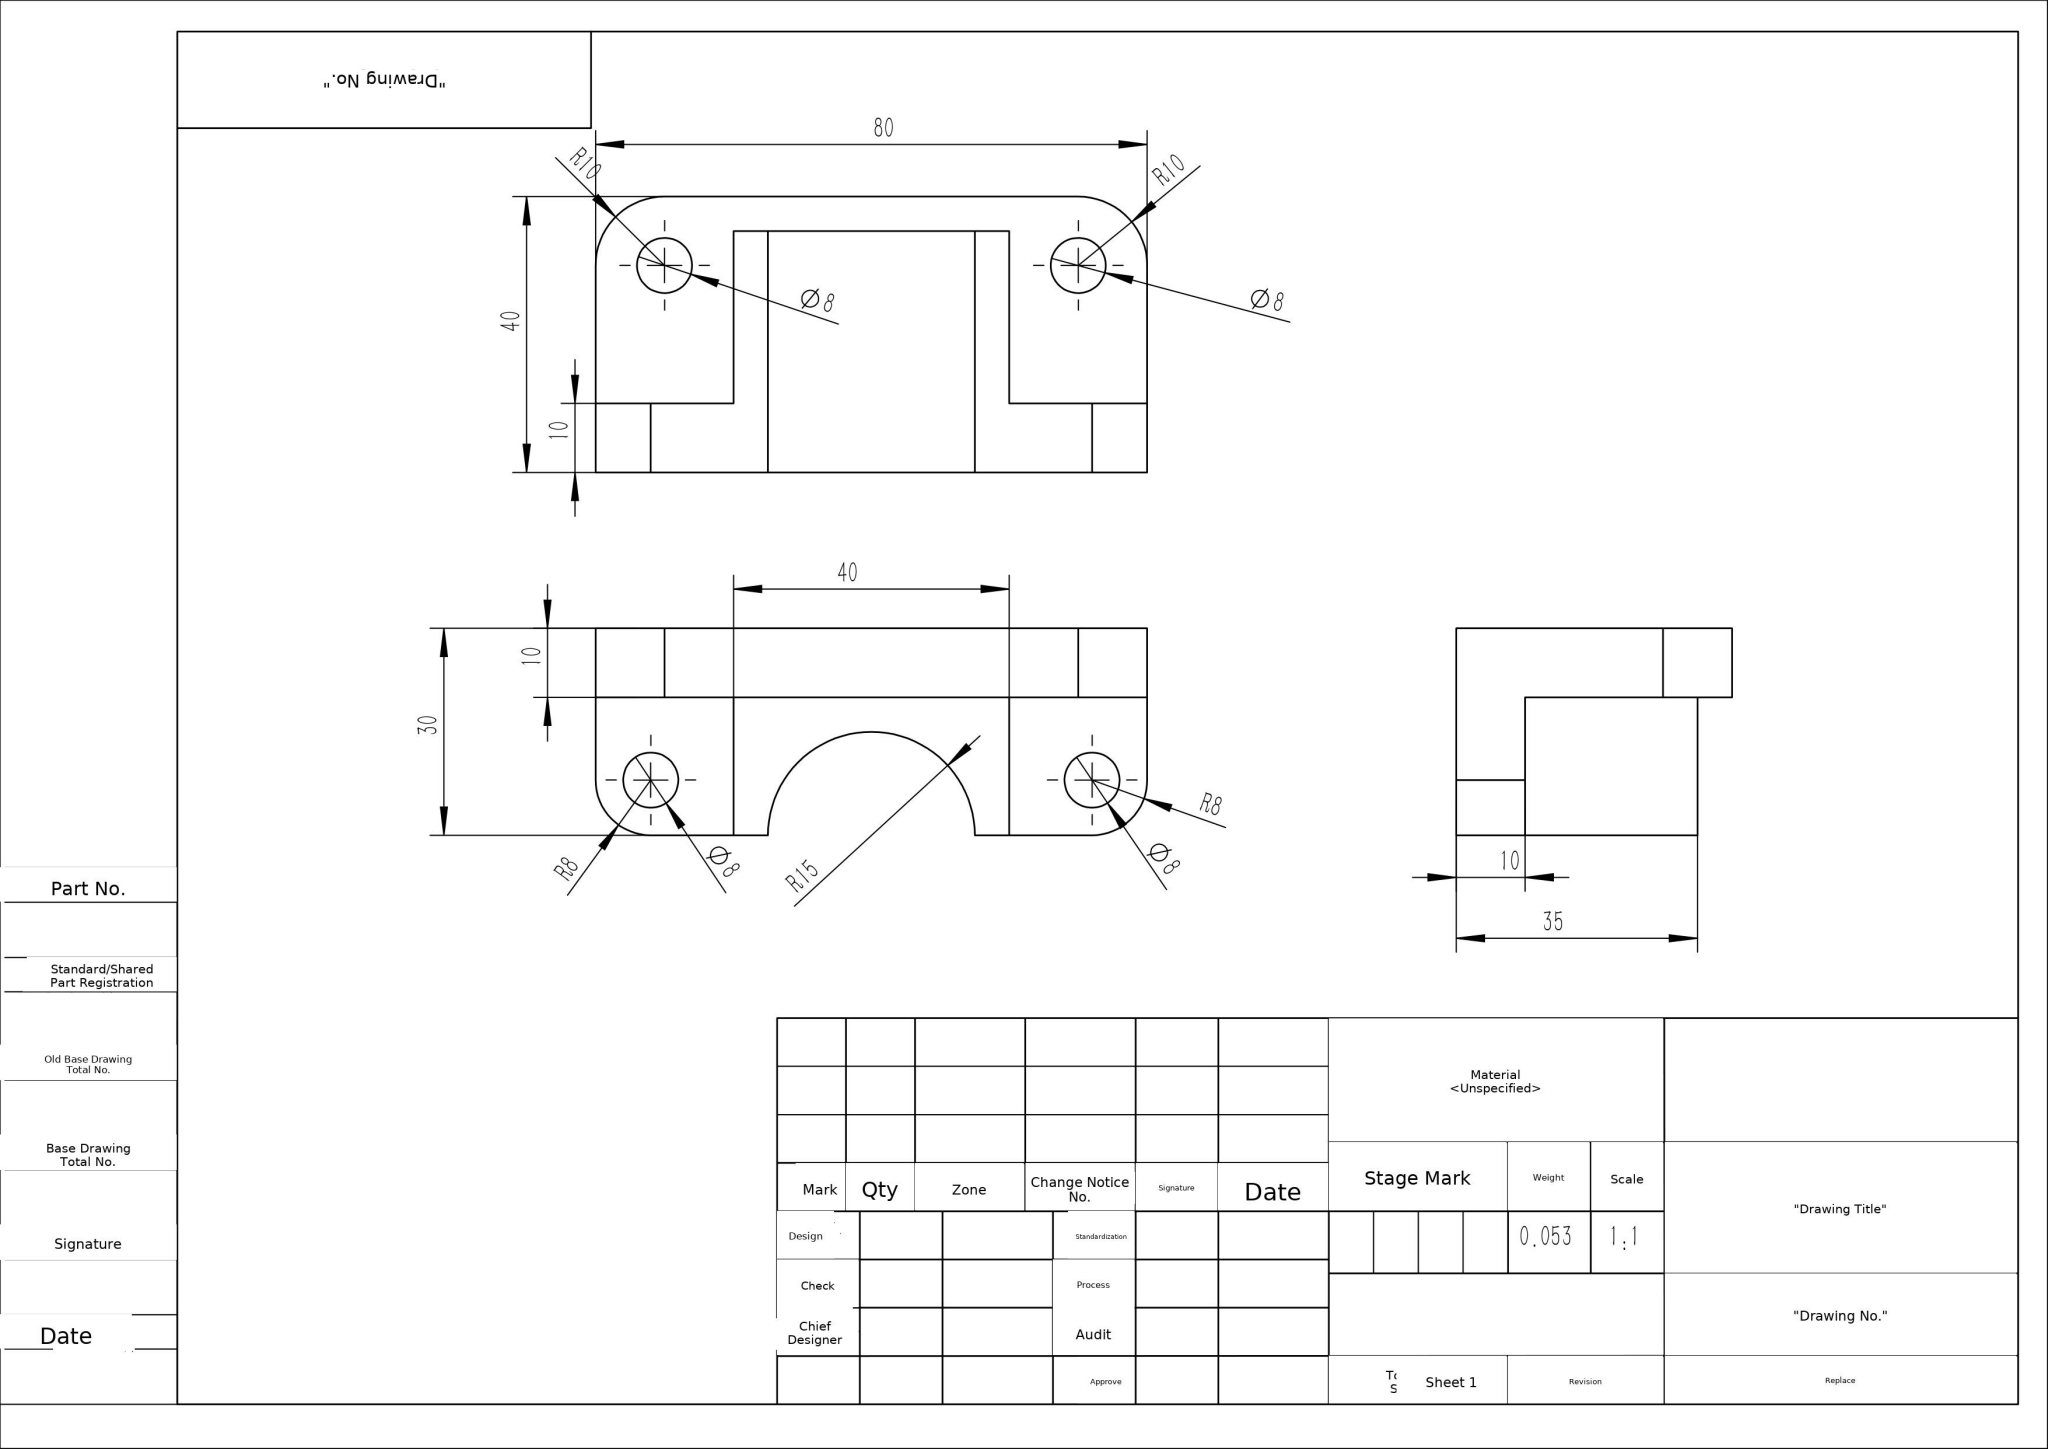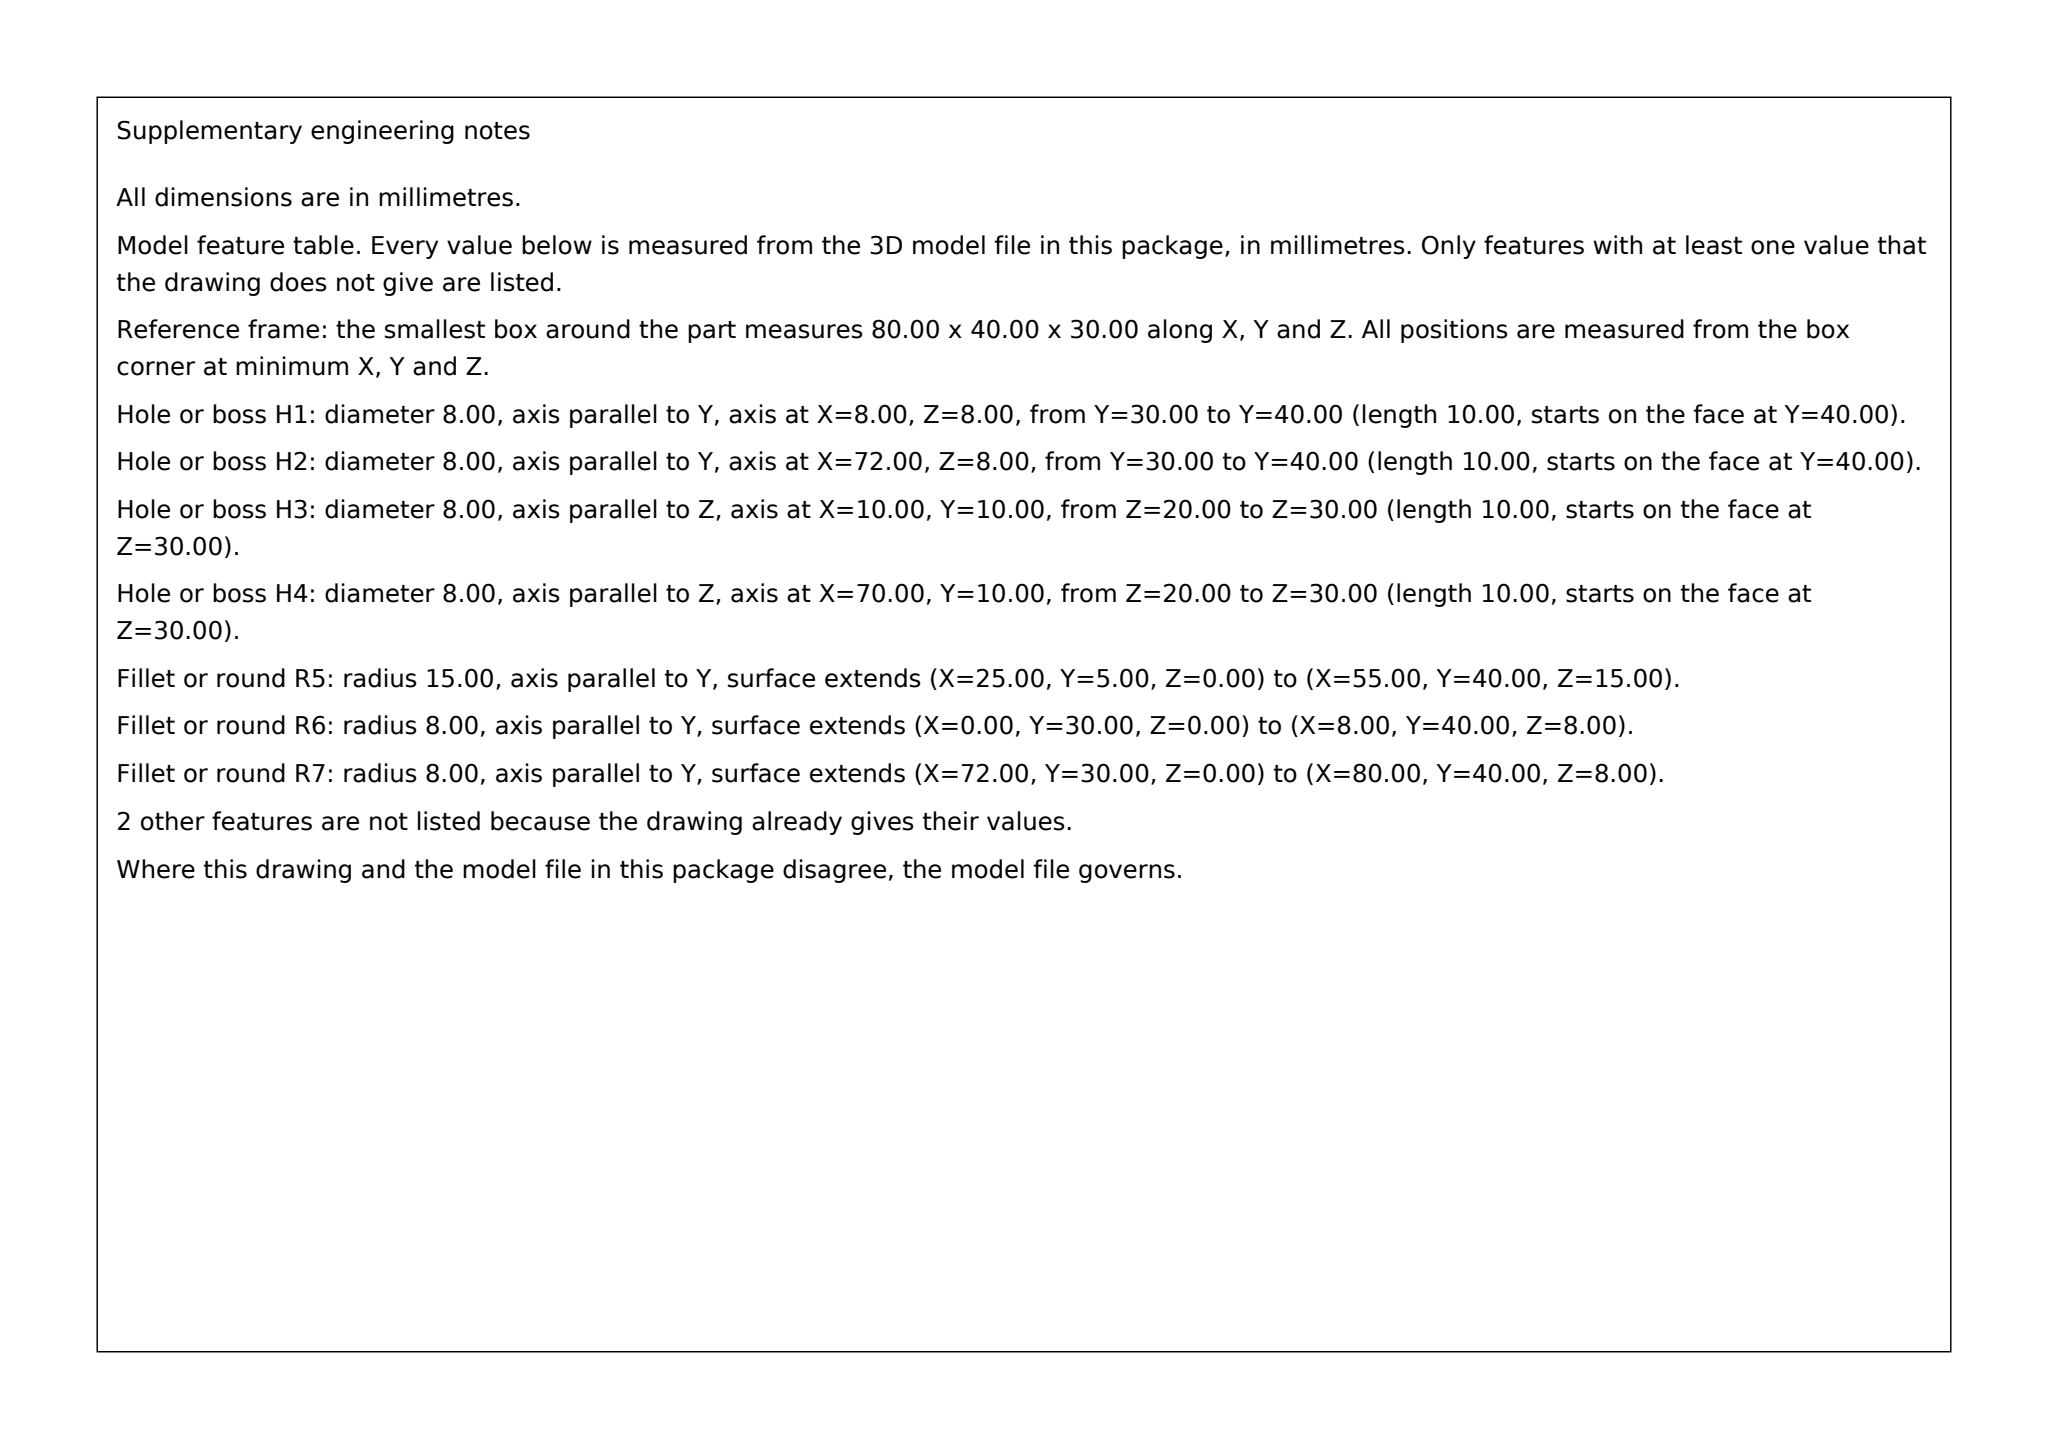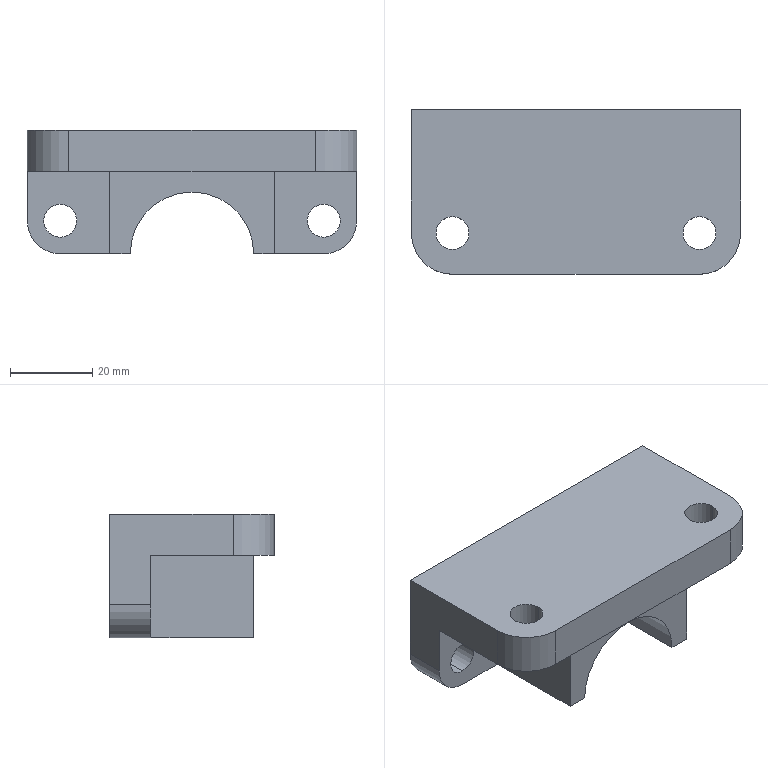Part | SolidWorks | mm | 1 solid | 27 faces | box 80 x 40 x 30 mm | volume 52915 mm3 | cylinder 14 | plane 13 | commonest cylinder face diameters 8 x8 30 x2 20 x2 16 x2
build123d program:
from build123d import *

# Parameters (mm, degrees)
SKETCH1_R           = 4
BOSS_EXTRUDE1_DEPTH = 10
SKETCH2_R           = 4
BOSS_EXTRUDE2_DEPTH = 10
BOSS_EXTRUDE3_DEPTH = 25


with BuildPart() as part:
    # Sketch1 → Boss-Extrude1 (new body)
    with BuildSketch(Plane.XY):
        with BuildLine():
            Line((-30, -20), (30, -20))
            ThreePointArc((30, -20), (37.071, -17.071), (40, -10))
            Line((40, -10), (40, 20))
            Line((40, 20), (-40, 20))
            Line((-40, 20), (-40, -10))
            ThreePointArc((-40, -10), (-37.071, -17.071), (-30, -20))
        make_face()
        with Locations((30, -10)):
            Circle(SKETCH1_R, mode=Mode.SUBTRACT)
        with Locations((-30, -10)):
            Circle(SKETCH1_R, mode=Mode.SUBTRACT)
    extrude(amount=BOSS_EXTRUDE1_DEPTH)

    # Sketch2 → Boss-Extrude2 (add)
    with BuildSketch(Plane(origin=(0, 20, 0), x_dir=(1, 0, 0), z_dir=(0, 1, 0))):
        with BuildLine():
            Line((15, 20), (32, 20))
            ThreePointArc((32, 20), (37.657, 17.657), (40, 12))
            Line((40, 12), (40, 0))
            Line((40, 0), (-40, 0))
            Line((-40, 0), (-40, 12))
            ThreePointArc((-40, 12), (-37.657, 17.657), (-32, 20))
            Line((-32, 20), (-15, 20))
            ThreePointArc((-15, 20), (0, 5), (15, 20))
        make_face()
        with Locations(Location((-32, 12, 0), (0, 0, 270))):
            Circle(SKETCH2_R, mode=Mode.SUBTRACT)
        with Locations(Location((32, 12, 0), (0, 0, 270))):
            Circle(SKETCH2_R, mode=Mode.SUBTRACT)
    extrude(amount=-BOSS_EXTRUDE2_DEPTH)

    # Sketch3 → Boss-Extrude3 (add)
    with BuildSketch(Plane.XZ.offset(-10)):
        with BuildLine():
            Line((-15, -20), (-20, -20))
            Line((-20, -20), (-20, 0))
            Line((-20, 0), (20, 0))
            Line((20, 0), (20, -20))
            Line((20, -20), (15, -20))
            ThreePointArc((15, -20), (0, -5), (-15, -20))
        make_face()
    extrude(amount=BOSS_EXTRUDE3_DEPTH)


solid = part.part
STEP:
#1=CARTESIAN_POINT('',(32.,10.,-16.));
#2=VERTEX_POINT('',#1);
#3=CARTESIAN_POINT('',(32.,10.,-8.));
#4=VERTEX_POINT('',#3);
#5=CARTESIAN_POINT('',(32.,10.,-12.));
#6=DIRECTION('',(0.,1.,0.));
#7=DIRECTION('',(0.,0.,1.));
#8=AXIS2_PLACEMENT_3D('',#5,#6,#7);
#9=CIRCLE('',#8,4.);
#10=EDGE_CURVE('',#2,#4,#9,.T.);
#11=ORIENTED_EDGE('',*,*,#10,.F.);
#12=CARTESIAN_POINT('',(32.,20.,-16.));
#13=VERTEX_POINT('',#12);
#14=CARTESIAN_POINT('',(32.,10.,-16.));
#15=DIRECTION('',(0.,1.,0.));
#16=VECTOR('',#15,1000.);
#17=LINE('',#14,#16);
#18=EDGE_CURVE('',#2,#13,#17,.T.);
#19=ORIENTED_EDGE('',*,*,#18,.T.);
#20=CARTESIAN_POINT('',(32.,20.,-8.));
#21=VERTEX_POINT('',#20);
#22=CARTESIAN_POINT('',(32.,20.,-12.));
#23=DIRECTION('',(0.,1.,0.));
#24=DIRECTION('',(0.,0.,1.));
#25=AXIS2_PLACEMENT_3D('',#22,#23,#24);
#26=CIRCLE('',#25,4.);
#27=EDGE_CURVE('',#13,#21,#26,.T.);
#28=ORIENTED_EDGE('',*,*,#27,.T.);
#29=CARTESIAN_POINT('',(32.,10.,-8.));
#30=DIRECTION('',(0.,1.,0.));
#31=VECTOR('',#30,1000.);
#32=LINE('',#29,#31);
#33=EDGE_CURVE('',#4,#21,#32,.T.);
#34=ORIENTED_EDGE('',*,*,#33,.F.);
#35=EDGE_LOOP('',(#11,#19,#28,#34));
#36=FACE_OUTER_BOUND('',#35,.T.);
#37=CARTESIAN_POINT('',(32.,10.,-12.));
#38=DIRECTION('',(0.,1.,0.));
#39=DIRECTION('',(0.,0.,1.));
#40=AXIS2_PLACEMENT_3D('',#37,#38,#39);
#41=CYLINDRICAL_SURFACE('',#40,4.);
#42=ADVANCED_FACE('',(#36),#41,.F.);
#43=CARTESIAN_POINT('',(-32.,10.,-16.));
#44=VERTEX_POINT('',#43);
#45=CARTESIAN_POINT('',(-32.,10.,-8.));
#46=VERTEX_POINT('',#45);
#47=CARTESIAN_POINT('',(-32.,10.,-12.));
#48=DIRECTION('',(0.,1.,0.));
#49=DIRECTION('',(0.,0.,1.));
#50=AXIS2_PLACEMENT_3D('',#47,#48,#49);
#51=CIRCLE('',#50,4.);
#52=EDGE_CURVE('',#44,#46,#51,.T.);
#53=ORIENTED_EDGE('',*,*,#52,.F.);
#54=CARTESIAN_POINT('',(-32.,20.,-16.));
#55=VERTEX_POINT('',#54);
#56=CARTESIAN_POINT('',(-32.,10.,-16.));
#57=DIRECTION('',(0.,1.,0.));
#58=VECTOR('',#57,1000.);
#59=LINE('',#56,#58);
#60=EDGE_CURVE('',#44,#55,#59,.T.);
#61=ORIENTED_EDGE('',*,*,#60,.T.);
#62=CARTESIAN_POINT('',(-32.,20.,-8.));
#63=VERTEX_POINT('',#62);
#64=CARTESIAN_POINT('',(-32.,20.,-12.));
#65=DIRECTION('',(0.,1.,0.));
#66=DIRECTION('',(0.,0.,1.));
#67=AXIS2_PLACEMENT_3D('',#64,#65,#66);
#68=CIRCLE('',#67,4.);
#69=EDGE_CURVE('',#55,#63,#68,.T.);
#70=ORIENTED_EDGE('',*,*,#69,.T.);
#71=CARTESIAN_POINT('',(-32.,10.,-8.));
#72=DIRECTION('',(0.,1.,0.));
#73=VECTOR('',#72,1000.);
#74=LINE('',#71,#73);
#75=EDGE_CURVE('',#46,#63,#74,.T.);
#76=ORIENTED_EDGE('',*,*,#75,.F.);
#77=EDGE_LOOP('',(#53,#61,#70,#76));
#78=FACE_OUTER_BOUND('',#77,.T.);
#79=CARTESIAN_POINT('',(-32.,10.,-12.));
#80=DIRECTION('',(0.,1.,0.));
#81=DIRECTION('',(0.,0.,1.));
#82=AXIS2_PLACEMENT_3D('',#79,#80,#81);
#83=CYLINDRICAL_SURFACE('',#82,4.);
#84=ADVANCED_FACE('',(#78),#83,.F.);
#85=CARTESIAN_POINT('',(-0.,-15.,-5.));
#86=VERTEX_POINT('',#85);
#87=CARTESIAN_POINT('',(15.,-15.,-20.));
#88=VERTEX_POINT('',#87);
#89=CARTESIAN_POINT('',(-0.,-15.,-20.));
#90=DIRECTION('',(0.,1.,0.));
#91=DIRECTION('',(0.,0.,-1.));
#92=AXIS2_PLACEMENT_3D('',#89,#90,#91);
#93=CIRCLE('',#92,15.);
#94=EDGE_CURVE('',#86,#88,#93,.T.);
#95=ORIENTED_EDGE('',*,*,#94,.F.);
#96=CARTESIAN_POINT('',(-0.,20.,-5.));
#97=VERTEX_POINT('',#96);
#98=CARTESIAN_POINT('',(-0.,10.,-5.));
#99=DIRECTION('',(0.,1.,0.));
#100=VECTOR('',#99,1000.);
#101=LINE('',#98,#100);
#102=EDGE_CURVE('',#86,#97,#101,.T.);
#103=ORIENTED_EDGE('',*,*,#102,.T.);
#104=CARTESIAN_POINT('',(15.,20.,-20.));
#105=VERTEX_POINT('',#104);
#106=CARTESIAN_POINT('',(-0.,20.,-20.));
#107=DIRECTION('',(0.,-1.,0.));
#108=DIRECTION('',(0.,0.,1.));
#109=AXIS2_PLACEMENT_3D('',#106,#107,#108);
#110=CIRCLE('',#109,15.);
#111=EDGE_CURVE('',#105,#97,#110,.T.);
#112=ORIENTED_EDGE('',*,*,#111,.F.);
#113=CARTESIAN_POINT('',(15.,10.,-20.));
#114=DIRECTION('',(0.,1.,0.));
#115=VECTOR('',#114,1000.);
#116=LINE('',#113,#115);
#117=EDGE_CURVE('',#88,#105,#116,.T.);
#118=ORIENTED_EDGE('',*,*,#117,.F.);
#119=EDGE_LOOP('',(#95,#103,#112,#118));
#120=FACE_OUTER_BOUND('',#119,.T.);
#121=CARTESIAN_POINT('',(-0.,10.,-20.));
#122=DIRECTION('',(0.,1.,0.));
#123=DIRECTION('',(0.,0.,1.));
#124=AXIS2_PLACEMENT_3D('',#121,#122,#123);
#125=CYLINDRICAL_SURFACE('',#124,15.);
#126=ADVANCED_FACE('',(#120),#125,.F.);
#127=CARTESIAN_POINT('',(-34.,-10.,10.));
#128=VERTEX_POINT('',#127);
#129=CARTESIAN_POINT('',(-26.,-10.,10.));
#130=VERTEX_POINT('',#129);
#131=CARTESIAN_POINT('',(-30.,-10.,10.));
#132=DIRECTION('',(0.,0.,1.));
#133=DIRECTION('',(1.,0.,0.));
#134=AXIS2_PLACEMENT_3D('',#131,#132,#133);
#135=CIRCLE('',#134,4.);
#136=EDGE_CURVE('',#128,#130,#135,.T.);
#137=ORIENTED_EDGE('',*,*,#136,.T.);
#138=CARTESIAN_POINT('',(-26.,-10.,0.));
#139=VERTEX_POINT('',#138);
#140=CARTESIAN_POINT('',(-26.,-10.,10.));
#141=DIRECTION('',(0.,0.,-1.));
#142=VECTOR('',#141,1000.);
#143=LINE('',#140,#142);
#144=EDGE_CURVE('',#130,#139,#143,.T.);
#145=ORIENTED_EDGE('',*,*,#144,.T.);
#146=CARTESIAN_POINT('',(-34.,-10.,0.));
#147=VERTEX_POINT('',#146);
#148=CARTESIAN_POINT('',(-30.,-10.,0.));
#149=DIRECTION('',(0.,0.,1.));
#150=DIRECTION('',(1.,0.,0.));
#151=AXIS2_PLACEMENT_3D('',#148,#149,#150);
#152=CIRCLE('',#151,4.);
#153=EDGE_CURVE('',#147,#139,#152,.T.);
#154=ORIENTED_EDGE('',*,*,#153,.F.);
#155=CARTESIAN_POINT('',(-34.,-10.,10.));
#156=DIRECTION('',(0.,0.,-1.));
#157=VECTOR('',#156,1000.);
#158=LINE('',#155,#157);
#159=EDGE_CURVE('',#128,#147,#158,.T.);
#160=ORIENTED_EDGE('',*,*,#159,.F.);
#161=EDGE_LOOP('',(#137,#145,#154,#160));
#162=FACE_OUTER_BOUND('',#161,.T.);
#163=CARTESIAN_POINT('',(-30.,-10.,10.));
#164=DIRECTION('',(0.,0.,-1.));
#165=DIRECTION('',(-1.,0.,0.));
#166=AXIS2_PLACEMENT_3D('',#163,#164,#165);
#167=CYLINDRICAL_SURFACE('',#166,4.);
#168=ADVANCED_FACE('',(#162),#167,.F.);
#169=CARTESIAN_POINT('',(26.,-10.,10.));
#170=VERTEX_POINT('',#169);
#171=CARTESIAN_POINT('',(34.,-10.,10.));
#172=VERTEX_POINT('',#171);
#173=CARTESIAN_POINT('',(30.,-10.,10.));
#174=DIRECTION('',(0.,0.,1.));
#175=DIRECTION('',(1.,0.,0.));
#176=AXIS2_PLACEMENT_3D('',#173,#174,#175);
#177=CIRCLE('',#176,4.);
#178=EDGE_CURVE('',#170,#172,#177,.T.);
#179=ORIENTED_EDGE('',*,*,#178,.T.);
#180=CARTESIAN_POINT('',(34.,-10.,0.));
#181=VERTEX_POINT('',#180);
#182=CARTESIAN_POINT('',(34.,-10.,10.));
#183=DIRECTION('',(0.,0.,-1.));
#184=VECTOR('',#183,1000.);
#185=LINE('',#182,#184);
#186=EDGE_CURVE('',#172,#181,#185,.T.);
#187=ORIENTED_EDGE('',*,*,#186,.T.);
#188=CARTESIAN_POINT('',(26.,-10.,0.));
#189=VERTEX_POINT('',#188);
#190=CARTESIAN_POINT('',(30.,-10.,0.));
#191=DIRECTION('',(0.,0.,1.));
#192=DIRECTION('',(1.,0.,0.));
#193=AXIS2_PLACEMENT_3D('',#190,#191,#192);
#194=CIRCLE('',#193,4.);
#195=EDGE_CURVE('',#189,#181,#194,.T.);
#196=ORIENTED_EDGE('',*,*,#195,.F.);
#197=CARTESIAN_POINT('',(26.,-10.,10.));
#198=DIRECTION('',(0.,0.,-1.));
#199=VECTOR('',#198,1000.);
#200=LINE('',#197,#199);
#201=EDGE_CURVE('',#170,#189,#200,.T.);
#202=ORIENTED_EDGE('',*,*,#201,.F.);
#203=EDGE_LOOP('',(#179,#187,#196,#202));
#204=FACE_OUTER_BOUND('',#203,.T.);
#205=CARTESIAN_POINT('',(30.,-10.,10.));
#206=DIRECTION('',(0.,0.,-1.));
#207=DIRECTION('',(-1.,0.,0.));
#208=AXIS2_PLACEMENT_3D('',#205,#206,#207);
#209=CYLINDRICAL_SURFACE('',#208,4.);
#210=ADVANCED_FACE('',(#204),#209,.F.);
#211=ORIENTED_EDGE('',*,*,#195,.T.);
#212=CARTESIAN_POINT('',(30.,-10.,0.));
#213=DIRECTION('',(0.,0.,1.));
#214=DIRECTION('',(1.,0.,0.));
#215=AXIS2_PLACEMENT_3D('',#212,#213,#214);
#216=CIRCLE('',#215,4.);
#217=EDGE_CURVE('',#181,#189,#216,.T.);
#218=ORIENTED_EDGE('',*,*,#217,.T.);
#219=EDGE_LOOP('',(#211,#218));
#220=FACE_BOUND('',#219,.T.);
#221=ORIENTED_EDGE('',*,*,#153,.T.);
#222=CARTESIAN_POINT('',(-30.,-10.,0.));
#223=DIRECTION('',(0.,0.,1.));
#224=DIRECTION('',(1.,0.,0.));
#225=AXIS2_PLACEMENT_3D('',#222,#223,#224);
#226=CIRCLE('',#225,4.);
#227=EDGE_CURVE('',#139,#147,#226,.T.);
#228=ORIENTED_EDGE('',*,*,#227,.T.);
#229=EDGE_LOOP('',(#221,#228));
#230=FACE_BOUND('',#229,.T.);
#231=CARTESIAN_POINT('',(20.,-15.,0.));
#232=VERTEX_POINT('',#231);
#233=CARTESIAN_POINT('',(-20.,-15.,-0.));
#234=VERTEX_POINT('',#233);
#235=CARTESIAN_POINT('',(-20.,-15.,-0.));
#236=DIRECTION('',(-1.,0.,-0.));
#237=VECTOR('',#236,1000.);
#238=LINE('',#235,#237);
#239=EDGE_CURVE('',#232,#234,#238,.T.);
#240=ORIENTED_EDGE('',*,*,#239,.F.);
#241=CARTESIAN_POINT('',(20.,10.,0.));
#242=VERTEX_POINT('',#241);
#243=CARTESIAN_POINT('',(20.,-15.,0.));
#244=DIRECTION('',(0.,1.,0.));
#245=VECTOR('',#244,1000.);
#246=LINE('',#243,#245);
#247=EDGE_CURVE('',#232,#242,#246,.T.);
#248=ORIENTED_EDGE('',*,*,#247,.T.);
#249=CARTESIAN_POINT('',(40.,10.,0.));
#250=VERTEX_POINT('',#249);
#251=CARTESIAN_POINT('',(-40.,10.,0.));
#252=DIRECTION('',(1.,0.,0.));
#253=VECTOR('',#252,1000.);
#254=LINE('',#251,#253);
#255=EDGE_CURVE('',#242,#250,#254,.T.);
#256=ORIENTED_EDGE('',*,*,#255,.T.);
#257=CARTESIAN_POINT('',(40.,-10.,0.));
#258=VERTEX_POINT('',#257);
#259=CARTESIAN_POINT('',(40.,-10.,0.));
#260=DIRECTION('',(0.,1.,0.));
#261=VECTOR('',#260,1000.);
#262=LINE('',#259,#261);
#263=EDGE_CURVE('',#258,#250,#262,.T.);
#264=ORIENTED_EDGE('',*,*,#263,.F.);
#265=CARTESIAN_POINT('',(30.,-20.,0.));
#266=VERTEX_POINT('',#265);
#267=CARTESIAN_POINT('',(30.,-10.,0.));
#268=DIRECTION('',(0.,0.,1.));
#269=DIRECTION('',(1.,0.,0.));
#270=AXIS2_PLACEMENT_3D('',#267,#268,#269);
#271=CIRCLE('',#270,10.);
#272=EDGE_CURVE('',#266,#258,#271,.T.);
#273=ORIENTED_EDGE('',*,*,#272,.F.);
#274=CARTESIAN_POINT('',(-30.,-20.,0.));
#275=VERTEX_POINT('',#274);
#276=CARTESIAN_POINT('',(-30.,-20.,0.));
#277=DIRECTION('',(1.,0.,0.));
#278=VECTOR('',#277,1000.);
#279=LINE('',#276,#278);
#280=EDGE_CURVE('',#275,#266,#279,.T.);
#281=ORIENTED_EDGE('',*,*,#280,.F.);
#282=CARTESIAN_POINT('',(-40.,-10.,0.));
#283=VERTEX_POINT('',#282);
#284=CARTESIAN_POINT('',(-30.,-10.,0.));
#285=DIRECTION('',(0.,0.,1.));
#286=DIRECTION('',(-1.,0.,0.));
#287=AXIS2_PLACEMENT_3D('',#284,#285,#286);
#288=CIRCLE('',#287,10.);
#289=EDGE_CURVE('',#283,#275,#288,.T.);
#290=ORIENTED_EDGE('',*,*,#289,.F.);
#291=CARTESIAN_POINT('',(-40.,10.,0.));
#292=VERTEX_POINT('',#291);
#293=CARTESIAN_POINT('',(-40.,-10.,0.));
#294=DIRECTION('',(0.,-1.,0.));
#295=VECTOR('',#294,1000.);
#296=LINE('',#293,#295);
#297=EDGE_CURVE('',#292,#283,#296,.T.);
#298=ORIENTED_EDGE('',*,*,#297,.F.);
#299=CARTESIAN_POINT('',(-20.,10.,-0.));
#300=VERTEX_POINT('',#299);
#301=CARTESIAN_POINT('',(-40.,10.,0.));
#302=DIRECTION('',(1.,0.,0.));
#303=VECTOR('',#302,1000.);
#304=LINE('',#301,#303);
#305=EDGE_CURVE('',#292,#300,#304,.T.);
#306=ORIENTED_EDGE('',*,*,#305,.T.);
#307=CARTESIAN_POINT('',(-20.,-15.,-0.));
#308=DIRECTION('',(0.,1.,0.));
#309=VECTOR('',#308,1000.);
#310=LINE('',#307,#309);
#311=EDGE_CURVE('',#234,#300,#310,.T.);
#312=ORIENTED_EDGE('',*,*,#311,.F.);
#313=EDGE_LOOP('',(#240,#248,#256,#264,#273,#281,#290,#298,#306,#312));
#314=FACE_OUTER_BOUND('',#313,.T.);
#315=CARTESIAN_POINT('',(-30.,-10.,0.));
#316=DIRECTION('',(0.,0.,-1.));
#317=DIRECTION('',(-1.,0.,0.));
#318=AXIS2_PLACEMENT_3D('',#315,#316,#317);
#319=PLANE('',#318);
#320=ADVANCED_FACE('',(#220,#230,#314),#319,.T.);
#321=CARTESIAN_POINT('',(32.,10.,-12.));
#322=DIRECTION('',(0.,1.,0.));
#323=DIRECTION('',(0.,0.,1.));
#324=AXIS2_PLACEMENT_3D('',#321,#322,#323);
#325=CIRCLE('',#324,4.);
#326=EDGE_CURVE('',#4,#2,#325,.T.);
#327=ORIENTED_EDGE('',*,*,#326,.T.);
#328=ORIENTED_EDGE('',*,*,#10,.T.);
#329=EDGE_LOOP('',(#327,#328));
#330=FACE_BOUND('',#329,.T.);
#331=ORIENTED_EDGE('',*,*,#255,.F.);
#332=CARTESIAN_POINT('',(20.,10.,-20.));
#333=VERTEX_POINT('',#332);
#334=CARTESIAN_POINT('',(20.,10.,0.));
#335=DIRECTION('',(0.,0.,1.));
#336=VECTOR('',#335,1000.);
#337=LINE('',#334,#336);
#338=EDGE_CURVE('',#333,#242,#337,.T.);
#339=ORIENTED_EDGE('',*,*,#338,.F.);
#340=CARTESIAN_POINT('',(32.,10.,-20.));
#341=VERTEX_POINT('',#340);
#342=CARTESIAN_POINT('',(15.,10.,-20.));
#343=DIRECTION('',(-1.,0.,0.));
#344=VECTOR('',#343,1000.);
#345=LINE('',#342,#344);
#346=EDGE_CURVE('',#341,#333,#345,.T.);
#347=ORIENTED_EDGE('',*,*,#346,.F.);
#348=CARTESIAN_POINT('',(40.,10.,-12.));
#349=VERTEX_POINT('',#348);
#350=CARTESIAN_POINT('',(32.,10.,-12.));
#351=DIRECTION('',(0.,1.,0.));
#352=DIRECTION('',(0.,0.,-1.));
#353=AXIS2_PLACEMENT_3D('',#350,#351,#352);
#354=CIRCLE('',#353,8.);
#355=EDGE_CURVE('',#349,#341,#354,.T.);
#356=ORIENTED_EDGE('',*,*,#355,.F.);
#357=CARTESIAN_POINT('',(40.,10.,0.));
#358=DIRECTION('',(0.,0.,-1.));
#359=VECTOR('',#358,1000.);
#360=LINE('',#357,#359);
#361=EDGE_CURVE('',#250,#349,#360,.T.);
#362=ORIENTED_EDGE('',*,*,#361,.F.);
#363=EDGE_LOOP('',(#331,#339,#347,#356,#362));
#364=FACE_OUTER_BOUND('',#363,.T.);
#365=CARTESIAN_POINT('',(-32.,10.,-12.));
#366=DIRECTION('',(0.,-1.,0.));
#367=DIRECTION('',(0.,0.,-1.));
#368=AXIS2_PLACEMENT_3D('',#365,#366,#367);
#369=PLANE('',#368);
#370=ADVANCED_FACE('',(#330,#364),#369,.T.);
#371=CARTESIAN_POINT('',(-32.,10.,-12.));
#372=DIRECTION('',(0.,1.,0.));
#373=DIRECTION('',(0.,0.,1.));
#374=AXIS2_PLACEMENT_3D('',#371,#372,#373);
#375=CIRCLE('',#374,4.);
#376=EDGE_CURVE('',#46,#44,#375,.T.);
#377=ORIENTED_EDGE('',*,*,#376,.T.);
#378=ORIENTED_EDGE('',*,*,#52,.T.);
#379=EDGE_LOOP('',(#377,#378));
#380=FACE_BOUND('',#379,.T.);
#381=CARTESIAN_POINT('',(-20.,10.,-20.));
#382=VERTEX_POINT('',#381);
#383=CARTESIAN_POINT('',(-32.,10.,-20.));
#384=VERTEX_POINT('',#383);
#385=CARTESIAN_POINT('',(-32.,10.,-20.));
#386=DIRECTION('',(-1.,0.,0.));
#387=VECTOR('',#386,1000.);
#388=LINE('',#385,#387);
#389=EDGE_CURVE('',#382,#384,#388,.T.);
#390=ORIENTED_EDGE('',*,*,#389,.F.);
#391=CARTESIAN_POINT('',(-20.,10.,-20.));
#392=DIRECTION('',(0.,0.,-1.));
#393=VECTOR('',#392,1000.);
#394=LINE('',#391,#393);
#395=EDGE_CURVE('',#300,#382,#394,.T.);
#396=ORIENTED_EDGE('',*,*,#395,.F.);
#397=ORIENTED_EDGE('',*,*,#305,.F.);
#398=CARTESIAN_POINT('',(-40.,10.,-12.));
#399=VERTEX_POINT('',#398);
#400=CARTESIAN_POINT('',(-40.,10.,0.));
#401=DIRECTION('',(0.,0.,1.));
#402=VECTOR('',#401,1000.);
#403=LINE('',#400,#402);
#404=EDGE_CURVE('',#399,#292,#403,.T.);
#405=ORIENTED_EDGE('',*,*,#404,.F.);
#406=CARTESIAN_POINT('',(-32.,10.,-12.));
#407=DIRECTION('',(0.,1.,0.));
#408=DIRECTION('',(0.,0.,-1.));
#409=AXIS2_PLACEMENT_3D('',#406,#407,#408);
#410=CIRCLE('',#409,8.);
#411=EDGE_CURVE('',#384,#399,#410,.T.);
#412=ORIENTED_EDGE('',*,*,#411,.F.);
#413=EDGE_LOOP('',(#390,#396,#397,#405,#412));
#414=FACE_OUTER_BOUND('',#413,.T.);
#415=CARTESIAN_POINT('',(-32.,10.,-12.));
#416=DIRECTION('',(0.,-1.,0.));
#417=DIRECTION('',(0.,0.,-1.));
#418=AXIS2_PLACEMENT_3D('',#415,#416,#417);
#419=PLANE('',#418);
#420=ADVANCED_FACE('',(#380,#414),#419,.T.);
#421=ORIENTED_EDGE('',*,*,#178,.F.);
#422=CARTESIAN_POINT('',(30.,-10.,10.));
#423=DIRECTION('',(0.,0.,1.));
#424=DIRECTION('',(1.,0.,0.));
#425=AXIS2_PLACEMENT_3D('',#422,#423,#424);
#426=CIRCLE('',#425,4.);
#427=EDGE_CURVE('',#172,#170,#426,.T.);
#428=ORIENTED_EDGE('',*,*,#427,.F.);
#429=EDGE_LOOP('',(#421,#428));
#430=FACE_BOUND('',#429,.T.);
#431=CARTESIAN_POINT('',(40.,-10.,10.));
#432=VERTEX_POINT('',#431);
#433=CARTESIAN_POINT('',(40.,20.,10.));
#434=VERTEX_POINT('',#433);
#435=CARTESIAN_POINT('',(40.,-10.,10.));
#436=DIRECTION('',(0.,1.,0.));
#437=VECTOR('',#436,1000.);
#438=LINE('',#435,#437);
#439=EDGE_CURVE('',#432,#434,#438,.T.);
#440=ORIENTED_EDGE('',*,*,#439,.T.);
#441=CARTESIAN_POINT('',(-40.,20.,10.));
#442=VERTEX_POINT('',#441);
#443=CARTESIAN_POINT('',(-40.,20.,10.));
#444=DIRECTION('',(-1.,0.,0.));
#445=VECTOR('',#444,1000.);
#446=LINE('',#443,#445);
#447=EDGE_CURVE('',#434,#442,#446,.T.);
#448=ORIENTED_EDGE('',*,*,#447,.T.);
#449=CARTESIAN_POINT('',(-40.,-10.,10.));
#450=VERTEX_POINT('',#449);
#451=CARTESIAN_POINT('',(-40.,-10.,10.));
#452=DIRECTION('',(0.,-1.,0.));
#453=VECTOR('',#452,1000.);
#454=LINE('',#451,#453);
#455=EDGE_CURVE('',#442,#450,#454,.T.);
#456=ORIENTED_EDGE('',*,*,#455,.T.);
#457=CARTESIAN_POINT('',(-30.,-20.,10.));
#458=VERTEX_POINT('',#457);
#459=CARTESIAN_POINT('',(-30.,-10.,10.));
#460=DIRECTION('',(0.,0.,1.));
#461=DIRECTION('',(-1.,0.,0.));
#462=AXIS2_PLACEMENT_3D('',#459,#460,#461);
#463=CIRCLE('',#462,10.);
#464=EDGE_CURVE('',#450,#458,#463,.T.);
#465=ORIENTED_EDGE('',*,*,#464,.T.);
#466=CARTESIAN_POINT('',(30.,-20.,10.));
#467=VERTEX_POINT('',#466);
#468=CARTESIAN_POINT('',(-30.,-20.,10.));
#469=DIRECTION('',(1.,0.,0.));
#470=VECTOR('',#469,1000.);
#471=LINE('',#468,#470);
#472=EDGE_CURVE('',#458,#467,#471,.T.);
#473=ORIENTED_EDGE('',*,*,#472,.T.);
#474=CARTESIAN_POINT('',(30.,-10.,10.));
#475=DIRECTION('',(0.,0.,1.));
#476=DIRECTION('',(1.,0.,0.));
#477=AXIS2_PLACEMENT_3D('',#474,#475,#476);
#478=CIRCLE('',#477,10.);
#479=EDGE_CURVE('',#467,#432,#478,.T.);
#480=ORIENTED_EDGE('',*,*,#479,.T.);
#481=EDGE_LOOP('',(#440,#448,#456,#465,#473,#480));
#482=FACE_OUTER_BOUND('',#481,.T.);
#483=ORIENTED_EDGE('',*,*,#136,.F.);
#484=CARTESIAN_POINT('',(-30.,-10.,10.));
#485=DIRECTION('',(0.,0.,1.));
#486=DIRECTION('',(1.,0.,0.));
#487=AXIS2_PLACEMENT_3D('',#484,#485,#486);
#488=CIRCLE('',#487,4.);
#489=EDGE_CURVE('',#130,#128,#488,.T.);
#490=ORIENTED_EDGE('',*,*,#489,.F.);
#491=EDGE_LOOP('',(#483,#490));
#492=FACE_BOUND('',#491,.T.);
#493=CARTESIAN_POINT('',(-30.,-10.,10.));
#494=DIRECTION('',(0.,0.,-1.));
#495=DIRECTION('',(-1.,0.,0.));
#496=AXIS2_PLACEMENT_3D('',#493,#494,#495);
#497=PLANE('',#496);
#498=ADVANCED_FACE('',(#430,#482,#492),#497,.F.);
#499=ORIENTED_EDGE('',*,*,#263,.T.);
#500=ORIENTED_EDGE('',*,*,#361,.T.);
#501=CARTESIAN_POINT('',(40.,20.,-12.));
#502=VERTEX_POINT('',#501);
#503=CARTESIAN_POINT('',(40.,10.,-12.));
#504=DIRECTION('',(0.,1.,0.));
#505=VECTOR('',#504,1000.);
#506=LINE('',#503,#505);
#507=EDGE_CURVE('',#349,#502,#506,.T.);
#508=ORIENTED_EDGE('',*,*,#507,.T.);
#509=CARTESIAN_POINT('',(40.,20.,10.));
#510=DIRECTION('',(0.,0.,-1.));
#511=VECTOR('',#510,1000.);
#512=LINE('',#509,#511);
#513=EDGE_CURVE('',#434,#502,#512,.T.);
#514=ORIENTED_EDGE('',*,*,#513,.F.);
#515=ORIENTED_EDGE('',*,*,#439,.F.);
#516=CARTESIAN_POINT('',(40.,-10.,10.));
#517=DIRECTION('',(0.,0.,-1.));
#518=VECTOR('',#517,1000.);
#519=LINE('',#516,#518);
#520=EDGE_CURVE('',#432,#258,#519,.T.);
#521=ORIENTED_EDGE('',*,*,#520,.T.);
#522=EDGE_LOOP('',(#499,#500,#508,#514,#515,#521));
#523=FACE_OUTER_BOUND('',#522,.T.);
#524=CARTESIAN_POINT('',(40.,-10.,10.));
#525=DIRECTION('',(-1.,0.,0.));
#526=DIRECTION('',(0.,0.,1.));
#527=AXIS2_PLACEMENT_3D('',#524,#525,#526);
#528=PLANE('',#527);
#529=ADVANCED_FACE('',(#523),#528,.F.);
#530=ORIENTED_EDGE('',*,*,#513,.T.);
#531=CARTESIAN_POINT('',(32.,20.,-20.));
#532=VERTEX_POINT('',#531);
#533=CARTESIAN_POINT('',(32.,20.,-12.));
#534=DIRECTION('',(0.,1.,0.));
#535=DIRECTION('',(0.,0.,-1.));
#536=AXIS2_PLACEMENT_3D('',#533,#534,#535);
#537=CIRCLE('',#536,8.);
#538=EDGE_CURVE('',#502,#532,#537,.T.);
#539=ORIENTED_EDGE('',*,*,#538,.T.);
#540=CARTESIAN_POINT('',(15.,20.,-20.));
#541=DIRECTION('',(-1.,0.,0.));
#542=VECTOR('',#541,1000.);
#543=LINE('',#540,#542);
#544=EDGE_CURVE('',#532,#105,#543,.T.);
#545=ORIENTED_EDGE('',*,*,#544,.T.);
#546=ORIENTED_EDGE('',*,*,#111,.T.);
#547=CARTESIAN_POINT('',(-15.,20.,-20.));
#548=VERTEX_POINT('',#547);
#549=CARTESIAN_POINT('',(-0.,20.,-20.));
#550=DIRECTION('',(0.,-1.,0.));
#551=DIRECTION('',(0.,0.,1.));
#552=AXIS2_PLACEMENT_3D('',#549,#550,#551);
#553=CIRCLE('',#552,15.);
#554=EDGE_CURVE('',#97,#548,#553,.T.);
#555=ORIENTED_EDGE('',*,*,#554,.T.);
#556=CARTESIAN_POINT('',(-32.,20.,-20.));
#557=VERTEX_POINT('',#556);
#558=CARTESIAN_POINT('',(-32.,20.,-20.));
#559=DIRECTION('',(-1.,0.,0.));
#560=VECTOR('',#559,1000.);
#561=LINE('',#558,#560);
#562=EDGE_CURVE('',#548,#557,#561,.T.);
#563=ORIENTED_EDGE('',*,*,#562,.T.);
#564=CARTESIAN_POINT('',(-40.,20.,-12.));
#565=VERTEX_POINT('',#564);
#566=CARTESIAN_POINT('',(-32.,20.,-12.));
#567=DIRECTION('',(0.,1.,0.));
#568=DIRECTION('',(0.,0.,-1.));
#569=AXIS2_PLACEMENT_3D('',#566,#567,#568);
#570=CIRCLE('',#569,8.);
#571=EDGE_CURVE('',#557,#565,#570,.T.);
#572=ORIENTED_EDGE('',*,*,#571,.T.);
#573=CARTESIAN_POINT('',(-40.,20.,10.));
#574=DIRECTION('',(0.,0.,-1.));
#575=VECTOR('',#574,1000.);
#576=LINE('',#573,#575);
#577=EDGE_CURVE('',#442,#565,#576,.T.);
#578=ORIENTED_EDGE('',*,*,#577,.F.);
#579=ORIENTED_EDGE('',*,*,#447,.F.);
#580=EDGE_LOOP('',(#530,#539,#545,#546,#555,#563,#572,#578,#579));
#581=FACE_OUTER_BOUND('',#580,.T.);
#582=CARTESIAN_POINT('',(32.,20.,-12.));
#583=DIRECTION('',(0.,1.,0.));
#584=DIRECTION('',(0.,0.,1.));
#585=AXIS2_PLACEMENT_3D('',#582,#583,#584);
#586=CIRCLE('',#585,4.);
#587=EDGE_CURVE('',#21,#13,#586,.T.);
#588=ORIENTED_EDGE('',*,*,#587,.F.);
#589=ORIENTED_EDGE('',*,*,#27,.F.);
#590=EDGE_LOOP('',(#588,#589));
#591=FACE_BOUND('',#590,.T.);
#592=CARTESIAN_POINT('',(-32.,20.,-12.));
#593=DIRECTION('',(0.,1.,0.));
#594=DIRECTION('',(0.,0.,1.));
#595=AXIS2_PLACEMENT_3D('',#592,#593,#594);
#596=CIRCLE('',#595,4.);
#597=EDGE_CURVE('',#63,#55,#596,.T.);
#598=ORIENTED_EDGE('',*,*,#597,.F.);
#599=ORIENTED_EDGE('',*,*,#69,.F.);
#600=EDGE_LOOP('',(#598,#599));
#601=FACE_BOUND('',#600,.T.);
#602=CARTESIAN_POINT('',(-40.,20.,10.));
#603=DIRECTION('',(0.,-1.,0.));
#604=DIRECTION('',(0.,0.,-1.));
#605=AXIS2_PLACEMENT_3D('',#602,#603,#604);
#606=PLANE('',#605);
#607=ADVANCED_FACE('',(#581,#591,#601),#606,.F.);
#608=ORIENTED_EDGE('',*,*,#577,.T.);
#609=CARTESIAN_POINT('',(-40.,10.,-12.));
#610=DIRECTION('',(0.,1.,0.));
#611=VECTOR('',#610,1000.);
#612=LINE('',#609,#611);
#613=EDGE_CURVE('',#399,#565,#612,.T.);
#614=ORIENTED_EDGE('',*,*,#613,.F.);
#615=ORIENTED_EDGE('',*,*,#404,.T.);
#616=ORIENTED_EDGE('',*,*,#297,.T.);
#617=CARTESIAN_POINT('',(-40.,-10.,10.));
#618=DIRECTION('',(0.,0.,-1.));
#619=VECTOR('',#618,1000.);
#620=LINE('',#617,#619);
#621=EDGE_CURVE('',#450,#283,#620,.T.);
#622=ORIENTED_EDGE('',*,*,#621,.F.);
#623=ORIENTED_EDGE('',*,*,#455,.F.);
#624=EDGE_LOOP('',(#608,#614,#615,#616,#622,#623));
#625=FACE_OUTER_BOUND('',#624,.T.);
#626=CARTESIAN_POINT('',(-40.,-10.,10.));
#627=DIRECTION('',(1.,0.,0.));
#628=DIRECTION('',(0.,0.,-1.));
#629=AXIS2_PLACEMENT_3D('',#626,#627,#628);
#630=PLANE('',#629);
#631=ADVANCED_FACE('',(#625),#630,.F.);
#632=ORIENTED_EDGE('',*,*,#289,.T.);
#633=CARTESIAN_POINT('',(-30.,-20.,10.));
#634=DIRECTION('',(0.,0.,-1.));
#635=VECTOR('',#634,1000.);
#636=LINE('',#633,#635);
#637=EDGE_CURVE('',#458,#275,#636,.T.);
#638=ORIENTED_EDGE('',*,*,#637,.F.);
#639=ORIENTED_EDGE('',*,*,#464,.F.);
#640=ORIENTED_EDGE('',*,*,#621,.T.);
#641=EDGE_LOOP('',(#632,#638,#639,#640));
#642=FACE_OUTER_BOUND('',#641,.T.);
#643=CARTESIAN_POINT('',(-30.,-10.,10.));
#644=DIRECTION('',(0.,0.,-1.));
#645=DIRECTION('',(-1.,0.,0.));
#646=AXIS2_PLACEMENT_3D('',#643,#644,#645);
#647=CYLINDRICAL_SURFACE('',#646,10.);
#648=ADVANCED_FACE('',(#642),#647,.T.);
#649=ORIENTED_EDGE('',*,*,#280,.T.);
#650=CARTESIAN_POINT('',(30.,-20.,10.));
#651=DIRECTION('',(0.,0.,-1.));
#652=VECTOR('',#651,1000.);
#653=LINE('',#650,#652);
#654=EDGE_CURVE('',#467,#266,#653,.T.);
#655=ORIENTED_EDGE('',*,*,#654,.F.);
#656=ORIENTED_EDGE('',*,*,#472,.F.);
#657=ORIENTED_EDGE('',*,*,#637,.T.);
#658=EDGE_LOOP('',(#649,#655,#656,#657));
#659=FACE_OUTER_BOUND('',#658,.T.);
#660=CARTESIAN_POINT('',(-30.,-20.,10.));
#661=DIRECTION('',(0.,1.,0.));
#662=DIRECTION('',(0.,0.,1.));
#663=AXIS2_PLACEMENT_3D('',#660,#661,#662);
#664=PLANE('',#663);
#665=ADVANCED_FACE('',(#659),#664,.F.);
#666=ORIENTED_EDGE('',*,*,#272,.T.);
#667=ORIENTED_EDGE('',*,*,#520,.F.);
#668=ORIENTED_EDGE('',*,*,#479,.F.);
#669=ORIENTED_EDGE('',*,*,#654,.T.);
#670=EDGE_LOOP('',(#666,#667,#668,#669));
#671=FACE_OUTER_BOUND('',#670,.T.);
#672=CARTESIAN_POINT('',(30.,-10.,10.));
#673=DIRECTION('',(0.,0.,-1.));
#674=DIRECTION('',(-1.,0.,0.));
#675=AXIS2_PLACEMENT_3D('',#672,#673,#674);
#676=CYLINDRICAL_SURFACE('',#675,10.);
#677=ADVANCED_FACE('',(#671),#676,.T.);
#678=ORIENTED_EDGE('',*,*,#186,.F.);
#679=ORIENTED_EDGE('',*,*,#427,.T.);
#680=ORIENTED_EDGE('',*,*,#201,.T.);
#681=ORIENTED_EDGE('',*,*,#217,.F.);
#682=EDGE_LOOP('',(#678,#679,#680,#681));
#683=FACE_OUTER_BOUND('',#682,.T.);
#684=CARTESIAN_POINT('',(30.,-10.,10.));
#685=DIRECTION('',(0.,0.,-1.));
#686=DIRECTION('',(-1.,0.,0.));
#687=AXIS2_PLACEMENT_3D('',#684,#685,#686);
#688=CYLINDRICAL_SURFACE('',#687,4.);
#689=ADVANCED_FACE('',(#683),#688,.F.);
#690=ORIENTED_EDGE('',*,*,#144,.F.);
#691=ORIENTED_EDGE('',*,*,#489,.T.);
#692=ORIENTED_EDGE('',*,*,#159,.T.);
#693=ORIENTED_EDGE('',*,*,#227,.F.);
#694=EDGE_LOOP('',(#690,#691,#692,#693));
#695=FACE_OUTER_BOUND('',#694,.T.);
#696=CARTESIAN_POINT('',(-30.,-10.,10.));
#697=DIRECTION('',(0.,0.,-1.));
#698=DIRECTION('',(-1.,0.,0.));
#699=AXIS2_PLACEMENT_3D('',#696,#697,#698);
#700=CYLINDRICAL_SURFACE('',#699,4.);
#701=ADVANCED_FACE('',(#695),#700,.F.);
#702=ORIENTED_EDGE('',*,*,#571,.F.);
#703=CARTESIAN_POINT('',(-32.,10.,-20.));
#704=DIRECTION('',(0.,1.,0.));
#705=VECTOR('',#704,1000.);
#706=LINE('',#703,#705);
#707=EDGE_CURVE('',#384,#557,#706,.T.);
#708=ORIENTED_EDGE('',*,*,#707,.F.);
#709=ORIENTED_EDGE('',*,*,#411,.T.);
#710=ORIENTED_EDGE('',*,*,#613,.T.);
#711=EDGE_LOOP('',(#702,#708,#709,#710));
#712=FACE_OUTER_BOUND('',#711,.T.);
#713=CARTESIAN_POINT('',(-32.,10.,-12.));
#714=DIRECTION('',(0.,1.,0.));
#715=DIRECTION('',(0.,0.,1.));
#716=AXIS2_PLACEMENT_3D('',#713,#714,#715);
#717=CYLINDRICAL_SURFACE('',#716,8.);
#718=ADVANCED_FACE('',(#712),#717,.T.);
#719=ORIENTED_EDGE('',*,*,#562,.F.);
#720=CARTESIAN_POINT('',(-15.,-15.,-20.));
#721=VERTEX_POINT('',#720);
#722=CARTESIAN_POINT('',(-15.,10.,-20.));
#723=DIRECTION('',(0.,1.,0.));
#724=VECTOR('',#723,1000.);
#725=LINE('',#722,#724);
#726=EDGE_CURVE('',#721,#548,#725,.T.);
#727=ORIENTED_EDGE('',*,*,#726,.F.);
#728=CARTESIAN_POINT('',(-20.,-15.,-20.));
#729=VERTEX_POINT('',#728);
#730=CARTESIAN_POINT('',(-15.,-15.,-20.));
#731=DIRECTION('',(1.,0.,0.));
#732=VECTOR('',#731,1000.);
#733=LINE('',#730,#732);
#734=EDGE_CURVE('',#729,#721,#733,.T.);
#735=ORIENTED_EDGE('',*,*,#734,.F.);
#736=CARTESIAN_POINT('',(-20.,-15.,-20.));
#737=DIRECTION('',(0.,1.,0.));
#738=VECTOR('',#737,1000.);
#739=LINE('',#736,#738);
#740=EDGE_CURVE('',#729,#382,#739,.T.);
#741=ORIENTED_EDGE('',*,*,#740,.T.);
#742=ORIENTED_EDGE('',*,*,#389,.T.);
#743=ORIENTED_EDGE('',*,*,#707,.T.);
#744=EDGE_LOOP('',(#719,#727,#735,#741,#742,#743));
#745=FACE_OUTER_BOUND('',#744,.T.);
#746=CARTESIAN_POINT('',(-32.,10.,-20.));
#747=DIRECTION('',(0.,0.,-1.));
#748=DIRECTION('',(-1.,0.,0.));
#749=AXIS2_PLACEMENT_3D('',#746,#747,#748);
#750=PLANE('',#749);
#751=ADVANCED_FACE('',(#745),#750,.T.);
#752=ORIENTED_EDGE('',*,*,#102,.F.);
#753=CARTESIAN_POINT('',(-0.,-15.,-20.));
#754=DIRECTION('',(0.,1.,0.));
#755=DIRECTION('',(0.,0.,-1.));
#756=AXIS2_PLACEMENT_3D('',#753,#754,#755);
#757=CIRCLE('',#756,15.);
#758=EDGE_CURVE('',#721,#86,#757,.T.);
#759=ORIENTED_EDGE('',*,*,#758,.F.);
#760=ORIENTED_EDGE('',*,*,#726,.T.);
#761=ORIENTED_EDGE('',*,*,#554,.F.);
#762=EDGE_LOOP('',(#752,#759,#760,#761));
#763=FACE_OUTER_BOUND('',#762,.T.);
#764=CARTESIAN_POINT('',(-0.,10.,-20.));
#765=DIRECTION('',(0.,1.,0.));
#766=DIRECTION('',(0.,0.,1.));
#767=AXIS2_PLACEMENT_3D('',#764,#765,#766);
#768=CYLINDRICAL_SURFACE('',#767,15.);
#769=ADVANCED_FACE('',(#763),#768,.F.);
#770=ORIENTED_EDGE('',*,*,#544,.F.);
#771=CARTESIAN_POINT('',(32.,10.,-20.));
#772=DIRECTION('',(0.,1.,0.));
#773=VECTOR('',#772,1000.);
#774=LINE('',#771,#773);
#775=EDGE_CURVE('',#341,#532,#774,.T.);
#776=ORIENTED_EDGE('',*,*,#775,.F.);
#777=ORIENTED_EDGE('',*,*,#346,.T.);
#778=CARTESIAN_POINT('',(20.,-15.,-20.));
#779=VERTEX_POINT('',#778);
#780=CARTESIAN_POINT('',(20.,-15.,-20.));
#781=DIRECTION('',(0.,1.,0.));
#782=VECTOR('',#781,1000.);
#783=LINE('',#780,#782);
#784=EDGE_CURVE('',#779,#333,#783,.T.);
#785=ORIENTED_EDGE('',*,*,#784,.F.);
#786=CARTESIAN_POINT('',(20.,-15.,-20.));
#787=DIRECTION('',(1.,0.,0.));
#788=VECTOR('',#787,1000.);
#789=LINE('',#786,#788);
#790=EDGE_CURVE('',#88,#779,#789,.T.);
#791=ORIENTED_EDGE('',*,*,#790,.F.);
#792=ORIENTED_EDGE('',*,*,#117,.T.);
#793=EDGE_LOOP('',(#770,#776,#777,#785,#791,#792));
#794=FACE_OUTER_BOUND('',#793,.T.);
#795=CARTESIAN_POINT('',(15.,10.,-20.));
#796=DIRECTION('',(0.,0.,-1.));
#797=DIRECTION('',(-1.,0.,0.));
#798=AXIS2_PLACEMENT_3D('',#795,#796,#797);
#799=PLANE('',#798);
#800=ADVANCED_FACE('',(#794),#799,.T.);
#801=ORIENTED_EDGE('',*,*,#538,.F.);
#802=ORIENTED_EDGE('',*,*,#507,.F.);
#803=ORIENTED_EDGE('',*,*,#355,.T.);
#804=ORIENTED_EDGE('',*,*,#775,.T.);
#805=EDGE_LOOP('',(#801,#802,#803,#804));
#806=FACE_OUTER_BOUND('',#805,.T.);
#807=CARTESIAN_POINT('',(32.,10.,-12.));
#808=DIRECTION('',(0.,1.,0.));
#809=DIRECTION('',(0.,0.,1.));
#810=AXIS2_PLACEMENT_3D('',#807,#808,#809);
#811=CYLINDRICAL_SURFACE('',#810,8.);
#812=ADVANCED_FACE('',(#806),#811,.T.);
#813=ORIENTED_EDGE('',*,*,#60,.F.);
#814=ORIENTED_EDGE('',*,*,#376,.F.);
#815=ORIENTED_EDGE('',*,*,#75,.T.);
#816=ORIENTED_EDGE('',*,*,#597,.T.);
#817=EDGE_LOOP('',(#813,#814,#815,#816));
#818=FACE_OUTER_BOUND('',#817,.T.);
#819=CARTESIAN_POINT('',(-32.,10.,-12.));
#820=DIRECTION('',(0.,1.,0.));
#821=DIRECTION('',(0.,0.,1.));
#822=AXIS2_PLACEMENT_3D('',#819,#820,#821);
#823=CYLINDRICAL_SURFACE('',#822,4.);
#824=ADVANCED_FACE('',(#818),#823,.F.);
#825=ORIENTED_EDGE('',*,*,#18,.F.);
#826=ORIENTED_EDGE('',*,*,#326,.F.);
#827=ORIENTED_EDGE('',*,*,#33,.T.);
#828=ORIENTED_EDGE('',*,*,#587,.T.);
#829=EDGE_LOOP('',(#825,#826,#827,#828));
#830=FACE_OUTER_BOUND('',#829,.T.);
#831=CARTESIAN_POINT('',(32.,10.,-12.));
#832=DIRECTION('',(0.,1.,0.));
#833=DIRECTION('',(0.,0.,1.));
#834=AXIS2_PLACEMENT_3D('',#831,#832,#833);
#835=CYLINDRICAL_SURFACE('',#834,4.);
#836=ADVANCED_FACE('',(#830),#835,.F.);
#837=ORIENTED_EDGE('',*,*,#338,.T.);
#838=ORIENTED_EDGE('',*,*,#247,.F.);
#839=CARTESIAN_POINT('',(20.,-15.,0.));
#840=DIRECTION('',(0.,0.,1.));
#841=VECTOR('',#840,1000.);
#842=LINE('',#839,#841);
#843=EDGE_CURVE('',#779,#232,#842,.T.);
#844=ORIENTED_EDGE('',*,*,#843,.F.);
#845=ORIENTED_EDGE('',*,*,#784,.T.);
#846=EDGE_LOOP('',(#837,#838,#844,#845));
#847=FACE_OUTER_BOUND('',#846,.T.);
#848=CARTESIAN_POINT('',(20.,-15.,0.));
#849=DIRECTION('',(-1.,0.,0.));
#850=DIRECTION('',(0.,0.,1.));
#851=AXIS2_PLACEMENT_3D('',#848,#849,#850);
#852=PLANE('',#851);
#853=ADVANCED_FACE('',(#847),#852,.F.);
#854=ORIENTED_EDGE('',*,*,#395,.T.);
#855=ORIENTED_EDGE('',*,*,#740,.F.);
#856=CARTESIAN_POINT('',(-20.,-15.,-20.));
#857=DIRECTION('',(0.,0.,-1.));
#858=VECTOR('',#857,1000.);
#859=LINE('',#856,#858);
#860=EDGE_CURVE('',#234,#729,#859,.T.);
#861=ORIENTED_EDGE('',*,*,#860,.F.);
#862=ORIENTED_EDGE('',*,*,#311,.T.);
#863=EDGE_LOOP('',(#854,#855,#861,#862));
#864=FACE_OUTER_BOUND('',#863,.T.);
#865=CARTESIAN_POINT('',(-20.,-15.,-20.));
#866=DIRECTION('',(1.,0.,0.));
#867=DIRECTION('',(0.,0.,-1.));
#868=AXIS2_PLACEMENT_3D('',#865,#866,#867);
#869=PLANE('',#868);
#870=ADVANCED_FACE('',(#864),#869,.F.);
#871=ORIENTED_EDGE('',*,*,#758,.T.);
#872=ORIENTED_EDGE('',*,*,#94,.T.);
#873=ORIENTED_EDGE('',*,*,#790,.T.);
#874=ORIENTED_EDGE('',*,*,#843,.T.);
#875=ORIENTED_EDGE('',*,*,#239,.T.);
#876=ORIENTED_EDGE('',*,*,#860,.T.);
#877=ORIENTED_EDGE('',*,*,#734,.T.);
#878=EDGE_LOOP('',(#871,#872,#873,#874,#875,#876,#877));
#879=FACE_OUTER_BOUND('',#878,.T.);
#880=CARTESIAN_POINT('',(-0.,-15.,-20.));
#881=DIRECTION('',(0.,-1.,0.));
#882=DIRECTION('',(0.,0.,-1.));
#883=AXIS2_PLACEMENT_3D('',#880,#881,#882);
#884=PLANE('',#883);
#885=ADVANCED_FACE('',(#879),#884,.T.);
#886=CLOSED_SHELL('',(#42,#84,#126,#168,#210,#320,#370,#420,#498,#529,#607,#631,#648,#665,#677,#689,#701,#718,#751,#769,#800,#812,#824,#836,#853,#870,#885));
#887=MANIFOLD_SOLID_BREP('',#886);
#888=CARTESIAN_POINT('',(0.,0.,0.));
#889=DIRECTION('',(0.,0.,1.));
#890=DIRECTION('',(1.,0.,0.));
#891=AXIS2_PLACEMENT_3D('',#888,#889,#890);
#892=(LENGTH_UNIT()NAMED_UNIT(*)SI_UNIT(.MILLI.,.METRE.));
#893=UNCERTAINTY_MEASURE_WITH_UNIT(LENGTH_MEASURE(0.00001),#892,'','');
#894=(NAMED_UNIT(*)PLANE_ANGLE_UNIT()SI_UNIT($,.RADIAN.));
#895=(NAMED_UNIT(*)SI_UNIT($,.STERADIAN.)SOLID_ANGLE_UNIT());
#896=(GEOMETRIC_REPRESENTATION_CONTEXT(3)GLOBAL_UNCERTAINTY_ASSIGNED_CONTEXT((#893))GLOBAL_UNIT_ASSIGNED_CONTEXT((#892,#894,#895))REPRESENTATION_CONTEXT('',''));
#897=ADVANCED_BREP_SHAPE_REPRESENTATION('',(#887,#891),#896);